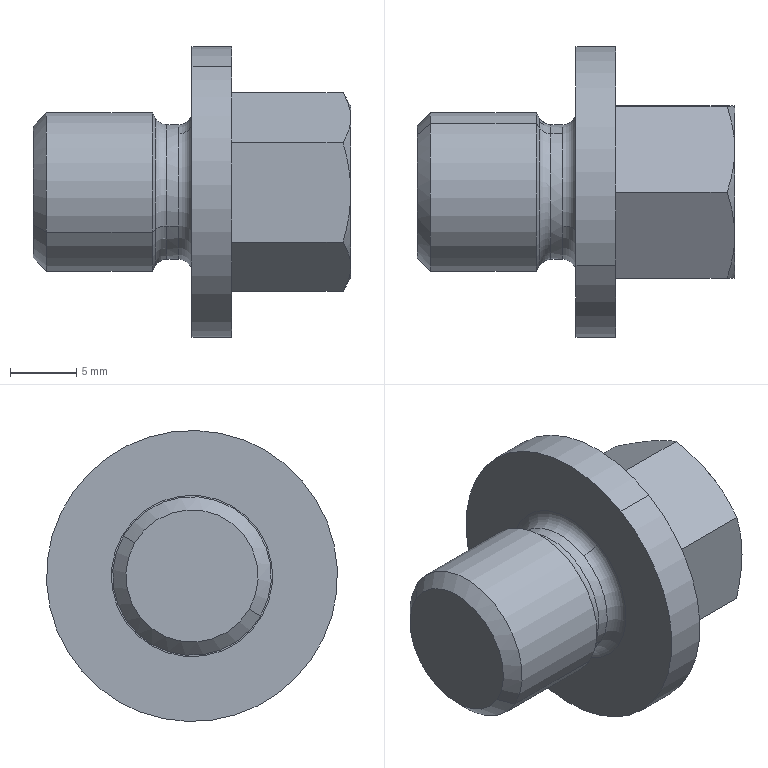Component | SolidWorks | JB_ZQ4450-1997[ExternalHexPlugM12_1.25]-1 | 1 solid | 30 faces | box 24 x 22 x 22 mm | volume 3717 mm3 | cone 10 | plane 10 | cylinder 6 | torus 4 | commonest cylinder face diameters 10.2 x2 12 x2 22 x2
STEP:
#1=COLOUR_RGB('',0.7922,0.8196,0.9333);
#2=FILL_AREA_STYLE_COLOUR('',#1);
#3=FILL_AREA_STYLE('',(#2));
#4=SURFACE_STYLE_FILL_AREA(#3);
#5=SURFACE_SIDE_STYLE('',(#4));
#6=SURFACE_STYLE_USAGE(.BOTH.,#5);
#7=PRESENTATION_STYLE_ASSIGNMENT((#6));
#8=CARTESIAN_POINT('',(7.835,-7.143,-0.1734));
#9=VERTEX_POINT('',#8);
#10=CARTESIAN_POINT('',(7.835,-7.417,-0.1013));
#11=VERTEX_POINT('',#10);
#12=CARTESIAN_POINT('',(7.835,-7.244,0.));
#13=DIRECTION('',(-1.,0.,0.));
#14=DIRECTION('',(0.,-0.5044,0.8635));
#15=AXIS2_PLACEMENT_3D('',#12,#13,#14);
#16=CIRCLE('',#15,0.2008);
#17=EDGE_CURVE('',#9,#11,#16,.T.);
#18=ORIENTED_EDGE('',*,*,#17,.F.);
#19=CARTESIAN_POINT('',(7.874,-7.123,-0.2074));
#20=VERTEX_POINT('',#19);
#21=CARTESIAN_POINT('',(7.835,-7.123,-0.2074));
#22=DIRECTION('',(0.,0.8635,0.5044));
#23=DIRECTION('',(0.,-0.5044,0.8635));
#24=AXIS2_PLACEMENT_3D('',#21,#22,#23);
#25=CIRCLE('',#24,0.03937);
#26=EDGE_CURVE('',#9,#20,#25,.T.);
#27=ORIENTED_EDGE('',*,*,#26,.T.);
#28=CARTESIAN_POINT('',(7.874,-7.365,0.2074));
#29=VERTEX_POINT('',#28);
#30=CARTESIAN_POINT('',(7.874,-7.244,0.));
#31=DIRECTION('',(1.,-0.,-0.));
#32=DIRECTION('',(0.,-0.5044,0.8635));
#33=AXIS2_PLACEMENT_3D('',#30,#31,#32);
#34=CIRCLE('',#33,0.2402);
#35=EDGE_CURVE('',#29,#20,#34,.T.);
#36=ORIENTED_EDGE('',*,*,#35,.F.);
#37=CARTESIAN_POINT('',(7.835,-7.345,0.1734));
#38=VERTEX_POINT('',#37);
#39=CARTESIAN_POINT('',(7.835,-7.365,0.2074));
#40=DIRECTION('',(-0.,-0.8635,-0.5044));
#41=DIRECTION('',(0.,0.5044,-0.8635));
#42=AXIS2_PLACEMENT_3D('',#39,#40,#41);
#43=CIRCLE('',#42,0.03937);
#44=EDGE_CURVE('',#38,#29,#43,.T.);
#45=ORIENTED_EDGE('',*,*,#44,.F.);
#46=CARTESIAN_POINT('',(7.835,-7.244,0.));
#47=DIRECTION('',(-1.,0.,0.));
#48=DIRECTION('',(0.,-0.5044,0.8635));
#49=AXIS2_PLACEMENT_3D('',#46,#47,#48);
#50=CIRCLE('',#49,0.2008);
#51=EDGE_CURVE('',#11,#38,#50,.T.);
#52=ORIENTED_EDGE('',*,*,#51,.F.);
#53=EDGE_LOOP('',(#18,#27,#36,#45,#52));
#54=FACE_OUTER_BOUND('',#53,.T.);
#55=CARTESIAN_POINT('',(7.835,-7.244,0.));
#56=DIRECTION('',(-1.,0.,0.));
#57=DIRECTION('',(-0.,-0.5044,0.8635));
#58=AXIS2_PLACEMENT_3D('',#55,#56,#57);
#59=TOROIDAL_SURFACE('',#58,0.2402,0.03937);
#60=ADVANCED_FACE('',(#54),#59,.F.);
#61=CARTESIAN_POINT('',(7.799,-7.417,-0.1013));
#62=VERTEX_POINT('',#61);
#63=CARTESIAN_POINT('',(7.799,-7.071,0.1013));
#64=VERTEX_POINT('',#63);
#65=CARTESIAN_POINT('',(7.799,-7.244,0.));
#66=DIRECTION('',(1.,-0.,0.));
#67=DIRECTION('',(0.,0.8635,0.5044));
#68=AXIS2_PLACEMENT_3D('',#65,#66,#67);
#69=CIRCLE('',#68,0.2008);
#70=EDGE_CURVE('',#62,#64,#69,.T.);
#71=ORIENTED_EDGE('',*,*,#70,.F.);
#72=CARTESIAN_POINT('',(7.765,-7.434,-0.1112));
#73=VERTEX_POINT('',#72);
#74=CARTESIAN_POINT('',(7.799,-7.451,-0.1211));
#75=DIRECTION('',(-0.,-0.5044,0.8635));
#76=DIRECTION('',(0.,-0.8635,-0.5044));
#77=AXIS2_PLACEMENT_3D('',#74,#75,#76);
#78=CIRCLE('',#77,0.03937);
#79=EDGE_CURVE('',#62,#73,#78,.T.);
#80=ORIENTED_EDGE('',*,*,#79,.T.);
#81=CARTESIAN_POINT('',(7.765,-7.054,0.1112));
#82=VERTEX_POINT('',#81);
#83=CARTESIAN_POINT('',(7.765,-7.244,0.));
#84=DIRECTION('',(-1.,0.,-0.));
#85=DIRECTION('',(0.,-0.8635,-0.5044));
#86=AXIS2_PLACEMENT_3D('',#83,#84,#85);
#87=CIRCLE('',#86,0.2205);
#88=EDGE_CURVE('',#82,#73,#87,.T.);
#89=ORIENTED_EDGE('',*,*,#88,.F.);
#90=CARTESIAN_POINT('',(7.799,-7.037,0.1211));
#91=DIRECTION('',(0.,0.5044,-0.8635));
#92=DIRECTION('',(0.,0.8635,0.5044));
#93=AXIS2_PLACEMENT_3D('',#90,#91,#92);
#94=CIRCLE('',#93,0.03937);
#95=EDGE_CURVE('',#64,#82,#94,.T.);
#96=ORIENTED_EDGE('',*,*,#95,.F.);
#97=EDGE_LOOP('',(#71,#80,#89,#96));
#98=FACE_OUTER_BOUND('',#97,.T.);
#99=CARTESIAN_POINT('',(7.799,-7.244,0.));
#100=DIRECTION('',(1.,-0.,0.));
#101=DIRECTION('',(0.,0.8635,0.5044));
#102=AXIS2_PLACEMENT_3D('',#99,#100,#101);
#103=TOROIDAL_SURFACE('',#102,0.2402,0.03937);
#104=ADVANCED_FACE('',(#98),#103,.F.);
#105=CARTESIAN_POINT('',(7.799,-7.244,0.));
#106=DIRECTION('',(1.,-0.,0.));
#107=DIRECTION('',(0.,0.8635,0.5044));
#108=AXIS2_PLACEMENT_3D('',#105,#106,#107);
#109=CIRCLE('',#108,0.2008);
#110=EDGE_CURVE('',#64,#62,#109,.T.);
#111=ORIENTED_EDGE('',*,*,#110,.T.);
#112=CARTESIAN_POINT('',(8.346,-7.417,-0.1013));
#113=DIRECTION('',(1.,-0.,0.));
#114=VECTOR('',#113,39.37);
#115=LINE('',#112,#114);
#116=EDGE_CURVE('',#62,#11,#115,.T.);
#117=ORIENTED_EDGE('',*,*,#116,.T.);
#118=ORIENTED_EDGE('',*,*,#51,.T.);
#119=CARTESIAN_POINT('',(7.835,-7.071,0.1013));
#120=VERTEX_POINT('',#119);
#121=CARTESIAN_POINT('',(7.835,-7.244,0.));
#122=DIRECTION('',(-1.,0.,0.));
#123=DIRECTION('',(0.,-0.5044,0.8635));
#124=AXIS2_PLACEMENT_3D('',#121,#122,#123);
#125=CIRCLE('',#124,0.2008);
#126=EDGE_CURVE('',#38,#120,#125,.T.);
#127=ORIENTED_EDGE('',*,*,#126,.T.);
#128=CARTESIAN_POINT('',(8.346,-7.071,0.1013));
#129=DIRECTION('',(1.,-0.,0.));
#130=VECTOR('',#129,39.37);
#131=LINE('',#128,#130);
#132=EDGE_CURVE('',#64,#120,#131,.T.);
#133=ORIENTED_EDGE('',*,*,#132,.F.);
#134=EDGE_LOOP('',(#111,#117,#118,#127,#133));
#135=FACE_OUTER_BOUND('',#134,.T.);
#136=CARTESIAN_POINT('',(8.346,-7.244,0.));
#137=DIRECTION('',(1.,-0.,0.));
#138=DIRECTION('',(0.,0.8635,0.5044));
#139=AXIS2_PLACEMENT_3D('',#136,#137,#138);
#140=CYLINDRICAL_SURFACE('',#139,0.2008);
#141=ADVANCED_FACE('',(#135),#140,.T.);
#142=CARTESIAN_POINT('',(7.765,-7.244,0.));
#143=DIRECTION('',(-1.,0.,-0.));
#144=DIRECTION('',(0.,-0.8635,-0.5044));
#145=AXIS2_PLACEMENT_3D('',#142,#143,#144);
#146=CIRCLE('',#145,0.2205);
#147=EDGE_CURVE('',#73,#82,#146,.T.);
#148=ORIENTED_EDGE('',*,*,#147,.T.);
#149=CARTESIAN_POINT('',(7.756,-7.04,0.1192));
#150=VERTEX_POINT('',#149);
#151=CARTESIAN_POINT('',(7.776,-7.071,0.1013));
#152=DIRECTION('',(-0.5,0.7478,0.4368));
#153=VECTOR('',#152,39.37);
#154=LINE('',#151,#153);
#155=EDGE_CURVE('',#82,#150,#154,.T.);
#156=ORIENTED_EDGE('',*,*,#155,.T.);
#157=CARTESIAN_POINT('',(7.756,-7.448,-0.1192));
#158=VERTEX_POINT('',#157);
#159=CARTESIAN_POINT('',(7.756,-7.244,0.));
#160=DIRECTION('',(1.,-0.,0.));
#161=DIRECTION('',(0.,0.8635,0.5044));
#162=AXIS2_PLACEMENT_3D('',#159,#160,#161);
#163=CIRCLE('',#162,0.2362);
#164=EDGE_CURVE('',#150,#158,#163,.T.);
#165=ORIENTED_EDGE('',*,*,#164,.T.);
#166=CARTESIAN_POINT('',(7.776,-7.417,-0.1013));
#167=DIRECTION('',(-0.5,-0.7478,-0.4368));
#168=VECTOR('',#167,39.37);
#169=LINE('',#166,#168);
#170=EDGE_CURVE('',#73,#158,#169,.T.);
#171=ORIENTED_EDGE('',*,*,#170,.F.);
#172=EDGE_LOOP('',(#148,#156,#165,#171));
#173=FACE_OUTER_BOUND('',#172,.T.);
#174=CARTESIAN_POINT('',(7.776,-7.244,0.));
#175=DIRECTION('',(-1.,0.,-0.));
#176=DIRECTION('',(0.,-0.8635,-0.5044));
#177=AXIS2_PLACEMENT_3D('',#174,#175,#176);
#178=CONICAL_SURFACE('',#177,0.2008,1.047);
#179=ADVANCED_FACE('',(#173),#178,.T.);
#180=CARTESIAN_POINT('',(7.441,-7.04,0.1192));
#181=VERTEX_POINT('',#180);
#182=CARTESIAN_POINT('',(7.441,-7.448,-0.1192));
#183=VERTEX_POINT('',#182);
#184=CARTESIAN_POINT('',(7.441,-7.244,0.));
#185=DIRECTION('',(1.,-0.,0.));
#186=DIRECTION('',(0.,0.8635,0.5044));
#187=AXIS2_PLACEMENT_3D('',#184,#185,#186);
#188=CIRCLE('',#187,0.2362);
#189=EDGE_CURVE('',#181,#183,#188,.T.);
#190=ORIENTED_EDGE('',*,*,#189,.T.);
#191=CARTESIAN_POINT('',(8.346,-7.448,-0.1192));
#192=DIRECTION('',(1.,-0.,0.));
#193=VECTOR('',#192,39.37);
#194=LINE('',#191,#193);
#195=EDGE_CURVE('',#183,#158,#194,.T.);
#196=ORIENTED_EDGE('',*,*,#195,.T.);
#197=ORIENTED_EDGE('',*,*,#164,.F.);
#198=CARTESIAN_POINT('',(8.346,-7.04,0.1192));
#199=DIRECTION('',(1.,-0.,0.));
#200=VECTOR('',#199,39.37);
#201=LINE('',#198,#200);
#202=EDGE_CURVE('',#181,#150,#201,.T.);
#203=ORIENTED_EDGE('',*,*,#202,.F.);
#204=EDGE_LOOP('',(#190,#196,#197,#203));
#205=FACE_OUTER_BOUND('',#204,.T.);
#206=CARTESIAN_POINT('',(8.346,-7.244,0.));
#207=DIRECTION('',(1.,-0.,0.));
#208=DIRECTION('',(0.,0.8635,0.5044));
#209=AXIS2_PLACEMENT_3D('',#206,#207,#208);
#210=CYLINDRICAL_SURFACE('',#209,0.2362);
#211=ADVANCED_FACE('',(#205),#210,.T.);
#212=CARTESIAN_POINT('',(7.402,-7.074,0.09929));
#213=VERTEX_POINT('',#212);
#214=CARTESIAN_POINT('',(7.402,-7.414,-0.09929));
#215=VERTEX_POINT('',#214);
#216=CARTESIAN_POINT('',(7.402,-7.244,0.));
#217=DIRECTION('',(1.,-0.,0.));
#218=DIRECTION('',(0.,0.8635,0.5044));
#219=AXIS2_PLACEMENT_3D('',#216,#217,#218);
#220=CIRCLE('',#219,0.1969);
#221=EDGE_CURVE('',#213,#215,#220,.T.);
#222=ORIENTED_EDGE('',*,*,#221,.T.);
#223=CARTESIAN_POINT('',(7.441,-7.448,-0.1192));
#224=DIRECTION('',(0.7071,-0.6106,-0.3567));
#225=VECTOR('',#224,39.37);
#226=LINE('',#223,#225);
#227=EDGE_CURVE('',#215,#183,#226,.T.);
#228=ORIENTED_EDGE('',*,*,#227,.T.);
#229=ORIENTED_EDGE('',*,*,#189,.F.);
#230=CARTESIAN_POINT('',(7.441,-7.04,0.1192));
#231=DIRECTION('',(0.7071,0.6106,0.3567));
#232=VECTOR('',#231,39.37);
#233=LINE('',#230,#232);
#234=EDGE_CURVE('',#213,#181,#233,.T.);
#235=ORIENTED_EDGE('',*,*,#234,.F.);
#236=EDGE_LOOP('',(#222,#228,#229,#235));
#237=FACE_OUTER_BOUND('',#236,.T.);
#238=CARTESIAN_POINT('',(7.441,-7.244,0.));
#239=DIRECTION('',(1.,-0.,0.));
#240=DIRECTION('',(0.,0.8635,0.5044));
#241=AXIS2_PLACEMENT_3D('',#238,#239,#240);
#242=CONICAL_SURFACE('',#241,0.2362,0.7854);
#243=ADVANCED_FACE('',(#237),#242,.T.);
#244=CARTESIAN_POINT('',(7.992,-7.463,0.3739));
#245=VERTEX_POINT('',#244);
#246=CARTESIAN_POINT('',(7.992,-7.026,-0.3739));
#247=VERTEX_POINT('',#246);
#248=CARTESIAN_POINT('',(7.992,-7.244,0.));
#249=DIRECTION('',(-1.,0.,0.));
#250=DIRECTION('',(0.,-0.5044,0.8635));
#251=AXIS2_PLACEMENT_3D('',#248,#249,#250);
#252=CIRCLE('',#251,0.4331);
#253=EDGE_CURVE('',#245,#247,#252,.T.);
#254=ORIENTED_EDGE('',*,*,#253,.T.);
#255=CARTESIAN_POINT('',(7.874,-7.026,-0.3739));
#256=VERTEX_POINT('',#255);
#257=CARTESIAN_POINT('',(7.992,-7.026,-0.3739));
#258=DIRECTION('',(-1.,0.,0.));
#259=VECTOR('',#258,39.37);
#260=LINE('',#257,#259);
#261=EDGE_CURVE('',#247,#256,#260,.T.);
#262=ORIENTED_EDGE('',*,*,#261,.T.);
#263=CARTESIAN_POINT('',(7.874,-7.463,0.3739));
#264=VERTEX_POINT('',#263);
#265=CARTESIAN_POINT('',(7.874,-7.244,0.));
#266=DIRECTION('',(-1.,0.,0.));
#267=DIRECTION('',(0.,-0.5044,0.8635));
#268=AXIS2_PLACEMENT_3D('',#265,#266,#267);
#269=CIRCLE('',#268,0.4331);
#270=EDGE_CURVE('',#264,#256,#269,.T.);
#271=ORIENTED_EDGE('',*,*,#270,.F.);
#272=CARTESIAN_POINT('',(7.992,-7.463,0.3739));
#273=DIRECTION('',(-1.,0.,0.));
#274=VECTOR('',#273,39.37);
#275=LINE('',#272,#274);
#276=EDGE_CURVE('',#245,#264,#275,.T.);
#277=ORIENTED_EDGE('',*,*,#276,.F.);
#278=EDGE_LOOP('',(#254,#262,#271,#277));
#279=FACE_OUTER_BOUND('',#278,.T.);
#280=CARTESIAN_POINT('',(7.992,-7.244,0.));
#281=DIRECTION('',(-1.,0.,0.));
#282=DIRECTION('',(0.,-0.5044,0.8635));
#283=AXIS2_PLACEMENT_3D('',#280,#281,#282);
#284=CYLINDRICAL_SURFACE('',#283,0.4331);
#285=ADVANCED_FACE('',(#279),#284,.T.);
#286=CARTESIAN_POINT('',(8.324,-6.989,0.1491));
#287=VERTEX_POINT('',#286);
#288=CARTESIAN_POINT('',(8.346,-7.117,0.2223));
#289=VERTEX_POINT('',#288);
#290=CARTESIAN_POINT('',(8.324,-6.989,0.1491));
#291=CARTESIAN_POINT('',(8.331,-7.01,0.161));
#292=CARTESIAN_POINT('',(8.336,-7.031,0.1731));
#293=CARTESIAN_POINT('',(8.344,-7.074,0.1975));
#294=CARTESIAN_POINT('',(8.346,-7.095,0.2098));
#295=CARTESIAN_POINT('',(8.346,-7.117,0.2223));
#296=B_SPLINE_CURVE_WITH_KNOTS('',3,(#290,#291,#292,#293,#294,#295),.UNSPECIFIED.,.F.,.F.,(4,2,4),(0.00000024,0.001899,0.003797),.UNSPECIFIED.);
#297=EDGE_CURVE('',#287,#289,#296,.T.);
#298=ORIENTED_EDGE('',*,*,#297,.F.);
#299=CARTESIAN_POINT('',(7.992,-6.989,0.1491));
#300=VERTEX_POINT('',#299);
#301=CARTESIAN_POINT('',(7.874,-6.989,0.1491));
#302=DIRECTION('',(1.,-0.,-0.));
#303=VECTOR('',#302,39.37);
#304=LINE('',#301,#303);
#305=EDGE_CURVE('',#300,#287,#304,.T.);
#306=ORIENTED_EDGE('',*,*,#305,.F.);
#307=CARTESIAN_POINT('',(7.992,-7.246,0.2955));
#308=VERTEX_POINT('',#307);
#309=CARTESIAN_POINT('',(7.992,-7.246,0.2955));
#310=DIRECTION('',(0.,0.8686,-0.4956));
#311=VECTOR('',#310,39.37);
#312=LINE('',#309,#311);
#313=EDGE_CURVE('',#308,#300,#312,.T.);
#314=ORIENTED_EDGE('',*,*,#313,.F.);
#315=CARTESIAN_POINT('',(8.324,-7.246,0.2955));
#316=VERTEX_POINT('',#315);
#317=CARTESIAN_POINT('',(7.874,-7.246,0.2955));
#318=DIRECTION('',(1.,-0.,-0.));
#319=VECTOR('',#318,39.37);
#320=LINE('',#317,#319);
#321=EDGE_CURVE('',#308,#316,#320,.T.);
#322=ORIENTED_EDGE('',*,*,#321,.T.);
#323=CARTESIAN_POINT('',(8.346,-7.117,0.2223));
#324=CARTESIAN_POINT('',(8.346,-7.128,0.2285));
#325=CARTESIAN_POINT('',(8.346,-7.139,0.2347));
#326=CARTESIAN_POINT('',(8.344,-7.161,0.2471));
#327=CARTESIAN_POINT('',(8.342,-7.171,0.2532));
#328=CARTESIAN_POINT('',(8.336,-7.204,0.2715));
#329=CARTESIAN_POINT('',(8.331,-7.225,0.2835));
#330=CARTESIAN_POINT('',(8.324,-7.246,0.2955));
#331=B_SPLINE_CURVE_WITH_KNOTS('',3,(#323,#324,#325,#326,#327,#328,#329,#330),.UNSPECIFIED.,.F.,.F.,(4,2,2,4),(0.003797,0.004743,0.005689,0.00758),.UNSPECIFIED.);
#332=EDGE_CURVE('',#289,#316,#331,.T.);
#333=ORIENTED_EDGE('',*,*,#332,.F.);
#334=EDGE_LOOP('',(#298,#306,#314,#322,#333));
#335=FACE_OUTER_BOUND('',#334,.T.);
#336=CARTESIAN_POINT('',(7.874,-7.246,0.2955));
#337=DIRECTION('',(-0.,-0.4956,-0.8686));
#338=DIRECTION('',(-0.,-0.8686,0.4956));
#339=AXIS2_PLACEMENT_3D('',#336,#337,#338);
#340=PLANE('',#339);
#341=ADVANCED_FACE('',(#335),#340,.F.);
#342=CARTESIAN_POINT('',(8.324,-6.987,-0.1464));
#343=VERTEX_POINT('',#342);
#344=CARTESIAN_POINT('',(8.346,-6.988,0.001305));
#345=VERTEX_POINT('',#344);
#346=CARTESIAN_POINT('',(8.324,-6.987,-0.1464));
#347=CARTESIAN_POINT('',(8.331,-6.988,-0.1223));
#348=CARTESIAN_POINT('',(8.336,-6.988,-0.09793));
#349=CARTESIAN_POINT('',(8.344,-6.988,-0.04872));
#350=CARTESIAN_POINT('',(8.346,-6.988,-0.02387));
#351=CARTESIAN_POINT('',(8.346,-6.988,0.001305));
#352=B_SPLINE_CURVE_WITH_KNOTS('',3,(#346,#347,#348,#349,#350,#351),.UNSPECIFIED.,.F.,.F.,(4,2,4),(0.00000024,0.001899,0.003797),.UNSPECIFIED.);
#353=EDGE_CURVE('',#343,#345,#352,.T.);
#354=ORIENTED_EDGE('',*,*,#353,.F.);
#355=CARTESIAN_POINT('',(7.992,-6.987,-0.1464));
#356=VERTEX_POINT('',#355);
#357=CARTESIAN_POINT('',(7.874,-6.987,-0.1464));
#358=DIRECTION('',(1.,-0.,-0.));
#359=VECTOR('',#358,39.37);
#360=LINE('',#357,#359);
#361=EDGE_CURVE('',#356,#343,#360,.T.);
#362=ORIENTED_EDGE('',*,*,#361,.F.);
#363=CARTESIAN_POINT('',(7.992,-6.989,0.1491));
#364=DIRECTION('',(-0.,0.005099,-1.));
#365=VECTOR('',#364,39.37);
#366=LINE('',#363,#365);
#367=EDGE_CURVE('',#300,#356,#366,.T.);
#368=ORIENTED_EDGE('',*,*,#367,.F.);
#369=ORIENTED_EDGE('',*,*,#305,.T.);
#370=CARTESIAN_POINT('',(8.346,-6.988,0.001305));
#371=CARTESIAN_POINT('',(8.346,-6.988,0.01384));
#372=CARTESIAN_POINT('',(8.346,-6.988,0.02644));
#373=CARTESIAN_POINT('',(8.344,-6.988,0.05135));
#374=CARTESIAN_POINT('',(8.342,-6.989,0.06373));
#375=CARTESIAN_POINT('',(8.336,-6.989,0.1006));
#376=CARTESIAN_POINT('',(8.331,-6.989,0.1249));
#377=CARTESIAN_POINT('',(8.324,-6.989,0.1491));
#378=B_SPLINE_CURVE_WITH_KNOTS('',3,(#370,#371,#372,#373,#374,#375,#376,#377),.UNSPECIFIED.,.F.,.F.,(4,2,2,4),(0.003797,0.004743,0.005689,0.00758),.UNSPECIFIED.);
#379=EDGE_CURVE('',#345,#287,#378,.T.);
#380=ORIENTED_EDGE('',*,*,#379,.F.);
#381=EDGE_LOOP('',(#354,#362,#368,#369,#380));
#382=FACE_OUTER_BOUND('',#381,.T.);
#383=CARTESIAN_POINT('',(7.874,-6.989,0.1491));
#384=DIRECTION('',(-0.,-1.,-0.005099));
#385=DIRECTION('',(0.,-0.005099,1.));
#386=AXIS2_PLACEMENT_3D('',#383,#384,#385);
#387=PLANE('',#386);
#388=ADVANCED_FACE('',(#382),#387,.F.);
#389=CARTESIAN_POINT('',(8.324,-7.243,-0.2955));
#390=VERTEX_POINT('',#389);
#391=CARTESIAN_POINT('',(8.346,-7.115,-0.221));
#392=VERTEX_POINT('',#391);
#393=CARTESIAN_POINT('',(8.324,-7.243,-0.2955));
#394=CARTESIAN_POINT('',(8.331,-7.222,-0.2833));
#395=CARTESIAN_POINT('',(8.336,-7.201,-0.2709));
#396=CARTESIAN_POINT('',(8.344,-7.158,-0.2461));
#397=CARTESIAN_POINT('',(8.346,-7.137,-0.2336));
#398=CARTESIAN_POINT('',(8.346,-7.115,-0.221));
#399=B_SPLINE_CURVE_WITH_KNOTS('',3,(#393,#394,#395,#396,#397,#398),.UNSPECIFIED.,.F.,.F.,(4,2,4),(0.007073,0.008973,0.01087),.UNSPECIFIED.);
#400=EDGE_CURVE('',#390,#392,#399,.T.);
#401=ORIENTED_EDGE('',*,*,#400,.F.);
#402=CARTESIAN_POINT('',(7.992,-7.243,-0.2955));
#403=VERTEX_POINT('',#402);
#404=CARTESIAN_POINT('',(7.874,-7.243,-0.2955));
#405=DIRECTION('',(1.,-0.,-0.));
#406=VECTOR('',#405,39.37);
#407=LINE('',#404,#406);
#408=EDGE_CURVE('',#403,#390,#407,.T.);
#409=ORIENTED_EDGE('',*,*,#408,.F.);
#410=CARTESIAN_POINT('',(7.992,-6.987,-0.1464));
#411=DIRECTION('',(-0.,-0.8635,-0.5044));
#412=VECTOR('',#411,39.37);
#413=LINE('',#410,#412);
#414=EDGE_CURVE('',#356,#403,#413,.T.);
#415=ORIENTED_EDGE('',*,*,#414,.F.);
#416=ORIENTED_EDGE('',*,*,#361,.T.);
#417=CARTESIAN_POINT('',(8.346,-7.115,-0.221));
#418=CARTESIAN_POINT('',(8.346,-7.104,-0.2147));
#419=CARTESIAN_POINT('',(8.346,-7.093,-0.2083));
#420=CARTESIAN_POINT('',(8.344,-7.072,-0.1956));
#421=CARTESIAN_POINT('',(8.342,-7.061,-0.1893));
#422=CARTESIAN_POINT('',(8.336,-7.029,-0.1707));
#423=CARTESIAN_POINT('',(8.331,-7.008,-0.1585));
#424=CARTESIAN_POINT('',(8.324,-6.987,-0.1464));
#425=B_SPLINE_CURVE_WITH_KNOTS('',3,(#417,#418,#419,#420,#421,#422,#423,#424),.UNSPECIFIED.,.F.,.F.,(4,2,2,4),(0.01087,0.01182,0.01277,0.01468),.UNSPECIFIED.);
#426=EDGE_CURVE('',#392,#343,#425,.T.);
#427=ORIENTED_EDGE('',*,*,#426,.F.);
#428=EDGE_LOOP('',(#401,#409,#415,#416,#427));
#429=FACE_OUTER_BOUND('',#428,.T.);
#430=CARTESIAN_POINT('',(7.874,-6.987,-0.1464));
#431=DIRECTION('',(-0.,-0.5044,0.8635));
#432=DIRECTION('',(0.,0.8635,0.5044));
#433=AXIS2_PLACEMENT_3D('',#430,#431,#432);
#434=PLANE('',#433);
#435=ADVANCED_FACE('',(#429),#434,.F.);
#436=CARTESIAN_POINT('',(8.324,-7.499,-0.1491));
#437=VERTEX_POINT('',#436);
#438=CARTESIAN_POINT('',(8.346,-7.371,-0.2223));
#439=VERTEX_POINT('',#438);
#440=CARTESIAN_POINT('',(8.324,-7.499,-0.1491));
#441=CARTESIAN_POINT('',(8.331,-7.478,-0.161));
#442=CARTESIAN_POINT('',(8.336,-7.457,-0.1731));
#443=CARTESIAN_POINT('',(8.344,-7.414,-0.1975));
#444=CARTESIAN_POINT('',(8.346,-7.393,-0.2098));
#445=CARTESIAN_POINT('',(8.346,-7.371,-0.2223));
#446=B_SPLINE_CURVE_WITH_KNOTS('',3,(#440,#441,#442,#443,#444,#445),.UNSPECIFIED.,.F.,.F.,(4,2,4),(0.00000024,0.001899,0.003797),.UNSPECIFIED.);
#447=EDGE_CURVE('',#437,#439,#446,.T.);
#448=ORIENTED_EDGE('',*,*,#447,.F.);
#449=CARTESIAN_POINT('',(7.992,-7.499,-0.1491));
#450=VERTEX_POINT('',#449);
#451=CARTESIAN_POINT('',(7.874,-7.499,-0.1491));
#452=DIRECTION('',(1.,-0.,-0.));
#453=VECTOR('',#452,39.37);
#454=LINE('',#451,#453);
#455=EDGE_CURVE('',#450,#437,#454,.T.);
#456=ORIENTED_EDGE('',*,*,#455,.F.);
#457=CARTESIAN_POINT('',(7.992,-7.243,-0.2955));
#458=DIRECTION('',(-0.,-0.8686,0.4956));
#459=VECTOR('',#458,39.37);
#460=LINE('',#457,#459);
#461=EDGE_CURVE('',#403,#450,#460,.T.);
#462=ORIENTED_EDGE('',*,*,#461,.F.);
#463=ORIENTED_EDGE('',*,*,#408,.T.);
#464=CARTESIAN_POINT('',(8.346,-7.371,-0.2223));
#465=CARTESIAN_POINT('',(8.346,-7.36,-0.2285));
#466=CARTESIAN_POINT('',(8.346,-7.349,-0.2347));
#467=CARTESIAN_POINT('',(8.344,-7.327,-0.2471));
#468=CARTESIAN_POINT('',(8.342,-7.317,-0.2532));
#469=CARTESIAN_POINT('',(8.336,-7.285,-0.2715));
#470=CARTESIAN_POINT('',(8.331,-7.264,-0.2835));
#471=CARTESIAN_POINT('',(8.324,-7.243,-0.2955));
#472=B_SPLINE_CURVE_WITH_KNOTS('',3,(#464,#465,#466,#467,#468,#469,#470,#471),.UNSPECIFIED.,.F.,.F.,(4,2,2,4),(0.003797,0.004743,0.005689,0.00758),.UNSPECIFIED.);
#473=EDGE_CURVE('',#439,#390,#472,.T.);
#474=ORIENTED_EDGE('',*,*,#473,.F.);
#475=EDGE_LOOP('',(#448,#456,#462,#463,#474));
#476=FACE_OUTER_BOUND('',#475,.T.);
#477=CARTESIAN_POINT('',(7.874,-7.243,-0.2955));
#478=DIRECTION('',(0.,0.4956,0.8686));
#479=DIRECTION('',(0.,0.8686,-0.4956));
#480=AXIS2_PLACEMENT_3D('',#477,#478,#479);
#481=PLANE('',#480);
#482=ADVANCED_FACE('',(#476),#481,.F.);
#483=CARTESIAN_POINT('',(8.324,-7.501,0.1464));
#484=VERTEX_POINT('',#483);
#485=CARTESIAN_POINT('',(8.346,-7.5,-0.001305));
#486=VERTEX_POINT('',#485);
#487=CARTESIAN_POINT('',(8.324,-7.501,0.1464));
#488=CARTESIAN_POINT('',(8.331,-7.501,0.1223));
#489=CARTESIAN_POINT('',(8.336,-7.501,0.09793));
#490=CARTESIAN_POINT('',(8.344,-7.5,0.04872));
#491=CARTESIAN_POINT('',(8.346,-7.5,0.02387));
#492=CARTESIAN_POINT('',(8.346,-7.5,-0.001305));
#493=B_SPLINE_CURVE_WITH_KNOTS('',3,(#487,#488,#489,#490,#491,#492),.UNSPECIFIED.,.F.,.F.,(4,2,4),(0.00000024,0.001899,0.003797),.UNSPECIFIED.);
#494=EDGE_CURVE('',#484,#486,#493,.T.);
#495=ORIENTED_EDGE('',*,*,#494,.F.);
#496=CARTESIAN_POINT('',(7.992,-7.501,0.1464));
#497=VERTEX_POINT('',#496);
#498=CARTESIAN_POINT('',(7.874,-7.501,0.1464));
#499=DIRECTION('',(1.,-0.,-0.));
#500=VECTOR('',#499,39.37);
#501=LINE('',#498,#500);
#502=EDGE_CURVE('',#497,#484,#501,.T.);
#503=ORIENTED_EDGE('',*,*,#502,.F.);
#504=CARTESIAN_POINT('',(7.992,-7.499,-0.1491));
#505=DIRECTION('',(0.,-0.005099,1.));
#506=VECTOR('',#505,39.37);
#507=LINE('',#504,#506);
#508=EDGE_CURVE('',#450,#497,#507,.T.);
#509=ORIENTED_EDGE('',*,*,#508,.F.);
#510=ORIENTED_EDGE('',*,*,#455,.T.);
#511=CARTESIAN_POINT('',(8.346,-7.5,-0.001305));
#512=CARTESIAN_POINT('',(8.346,-7.5,-0.01384));
#513=CARTESIAN_POINT('',(8.346,-7.5,-0.02644));
#514=CARTESIAN_POINT('',(8.344,-7.5,-0.05135));
#515=CARTESIAN_POINT('',(8.342,-7.5,-0.06373));
#516=CARTESIAN_POINT('',(8.336,-7.499,-0.1006));
#517=CARTESIAN_POINT('',(8.331,-7.499,-0.1249));
#518=CARTESIAN_POINT('',(8.324,-7.499,-0.1491));
#519=B_SPLINE_CURVE_WITH_KNOTS('',3,(#511,#512,#513,#514,#515,#516,#517,#518),.UNSPECIFIED.,.F.,.F.,(4,2,2,4),(0.003797,0.004743,0.005689,0.00758),.UNSPECIFIED.);
#520=EDGE_CURVE('',#486,#437,#519,.T.);
#521=ORIENTED_EDGE('',*,*,#520,.F.);
#522=EDGE_LOOP('',(#495,#503,#509,#510,#521));
#523=FACE_OUTER_BOUND('',#522,.T.);
#524=CARTESIAN_POINT('',(7.874,-7.499,-0.1491));
#525=DIRECTION('',(0.,1.,0.005099));
#526=DIRECTION('',(-0.,0.005099,-1.));
#527=AXIS2_PLACEMENT_3D('',#524,#525,#526);
#528=PLANE('',#527);
#529=ADVANCED_FACE('',(#523),#528,.F.);
#530=CARTESIAN_POINT('',(8.346,-7.373,0.221));
#531=VERTEX_POINT('',#530);
#532=CARTESIAN_POINT('',(8.324,-7.246,0.2955));
#533=CARTESIAN_POINT('',(8.331,-7.266,0.2834));
#534=CARTESIAN_POINT('',(8.336,-7.287,0.2712));
#535=CARTESIAN_POINT('',(8.342,-7.319,0.2526));
#536=CARTESIAN_POINT('',(8.344,-7.33,0.2463));
#537=CARTESIAN_POINT('',(8.346,-7.351,0.2336));
#538=CARTESIAN_POINT('',(8.346,-7.362,0.2273));
#539=CARTESIAN_POINT('',(8.346,-7.373,0.221));
#540=B_SPLINE_CURVE_WITH_KNOTS('',3,(#532,#533,#534,#535,#536,#537,#538,#539),.UNSPECIFIED.,.F.,.F.,(4,2,2,4),(0.01868,0.02058,0.02153,0.02248),.UNSPECIFIED.);
#541=EDGE_CURVE('',#316,#531,#540,.T.);
#542=ORIENTED_EDGE('',*,*,#541,.F.);
#543=ORIENTED_EDGE('',*,*,#321,.F.);
#544=CARTESIAN_POINT('',(7.992,-7.501,0.1464));
#545=DIRECTION('',(0.,0.8635,0.5044));
#546=VECTOR('',#545,39.37);
#547=LINE('',#544,#546);
#548=EDGE_CURVE('',#497,#308,#547,.T.);
#549=ORIENTED_EDGE('',*,*,#548,.F.);
#550=ORIENTED_EDGE('',*,*,#502,.T.);
#551=CARTESIAN_POINT('',(8.346,-7.373,0.221));
#552=CARTESIAN_POINT('',(8.346,-7.395,0.2083));
#553=CARTESIAN_POINT('',(8.344,-7.416,0.1958));
#554=CARTESIAN_POINT('',(8.336,-7.459,0.171));
#555=CARTESIAN_POINT('',(8.331,-7.48,0.1586));
#556=CARTESIAN_POINT('',(8.324,-7.501,0.1464));
#557=B_SPLINE_CURVE_WITH_KNOTS('',3,(#551,#552,#553,#554,#555,#556),.UNSPECIFIED.,.F.,.F.,(4,2,4),(0.02248,0.02438,0.02628),.UNSPECIFIED.);
#558=EDGE_CURVE('',#531,#484,#557,.T.);
#559=ORIENTED_EDGE('',*,*,#558,.F.);
#560=EDGE_LOOP('',(#542,#543,#549,#550,#559));
#561=FACE_OUTER_BOUND('',#560,.T.);
#562=CARTESIAN_POINT('',(7.874,-7.501,0.1464));
#563=DIRECTION('',(0.,0.5044,-0.8635));
#564=DIRECTION('',(-0.,-0.8635,-0.5044));
#565=AXIS2_PLACEMENT_3D('',#562,#563,#564);
#566=PLANE('',#565);
#567=ADVANCED_FACE('',(#561),#566,.F.);
#568=ORIENTED_EDGE('',*,*,#253,.F.);
#569=CARTESIAN_POINT('',(7.992,-7.244,0.));
#570=DIRECTION('',(-1.,0.,0.));
#571=DIRECTION('',(0.,-0.5044,0.8635));
#572=AXIS2_PLACEMENT_3D('',#569,#570,#571);
#573=CIRCLE('',#572,0.4331);
#574=EDGE_CURVE('',#247,#245,#573,.T.);
#575=ORIENTED_EDGE('',*,*,#574,.F.);
#576=EDGE_LOOP('',(#568,#575));
#577=FACE_OUTER_BOUND('',#576,.T.);
#578=ORIENTED_EDGE('',*,*,#548,.T.);
#579=ORIENTED_EDGE('',*,*,#313,.T.);
#580=ORIENTED_EDGE('',*,*,#367,.T.);
#581=ORIENTED_EDGE('',*,*,#414,.T.);
#582=ORIENTED_EDGE('',*,*,#461,.T.);
#583=ORIENTED_EDGE('',*,*,#508,.T.);
#584=EDGE_LOOP('',(#578,#579,#580,#581,#582,#583));
#585=FACE_BOUND('',#584,.T.);
#586=CARTESIAN_POINT('',(7.992,-7.244,0.));
#587=DIRECTION('',(-1.,0.,0.));
#588=DIRECTION('',(-0.,-0.5044,0.8635));
#589=AXIS2_PLACEMENT_3D('',#586,#587,#588);
#590=PLANE('',#589);
#591=ADVANCED_FACE('',(#577,#585),#590,.F.);
#592=ORIENTED_EDGE('',*,*,#261,.F.);
#593=ORIENTED_EDGE('',*,*,#574,.T.);
#594=ORIENTED_EDGE('',*,*,#276,.T.);
#595=CARTESIAN_POINT('',(7.874,-7.244,0.));
#596=DIRECTION('',(-1.,0.,0.));
#597=DIRECTION('',(0.,-0.5044,0.8635));
#598=AXIS2_PLACEMENT_3D('',#595,#596,#597);
#599=CIRCLE('',#598,0.4331);
#600=EDGE_CURVE('',#256,#264,#599,.T.);
#601=ORIENTED_EDGE('',*,*,#600,.F.);
#602=EDGE_LOOP('',(#592,#593,#594,#601));
#603=FACE_OUTER_BOUND('',#602,.T.);
#604=CARTESIAN_POINT('',(7.992,-7.244,0.));
#605=DIRECTION('',(-1.,0.,0.));
#606=DIRECTION('',(0.,-0.5044,0.8635));
#607=AXIS2_PLACEMENT_3D('',#604,#605,#606);
#608=CYLINDRICAL_SURFACE('',#607,0.4331);
#609=ADVANCED_FACE('',(#603),#608,.T.);
#610=ORIENTED_EDGE('',*,*,#35,.T.);
#611=CARTESIAN_POINT('',(7.874,-7.244,0.));
#612=DIRECTION('',(1.,-0.,-0.));
#613=DIRECTION('',(0.,-0.5044,0.8635));
#614=AXIS2_PLACEMENT_3D('',#611,#612,#613);
#615=CIRCLE('',#614,0.2402);
#616=EDGE_CURVE('',#20,#29,#615,.T.);
#617=ORIENTED_EDGE('',*,*,#616,.T.);
#618=EDGE_LOOP('',(#610,#617));
#619=FACE_BOUND('',#618,.T.);
#620=ORIENTED_EDGE('',*,*,#270,.T.);
#621=ORIENTED_EDGE('',*,*,#600,.T.);
#622=EDGE_LOOP('',(#620,#621));
#623=FACE_OUTER_BOUND('',#622,.T.);
#624=CARTESIAN_POINT('',(7.874,-6.732,0.00261));
#625=DIRECTION('',(-1.,0.,0.));
#626=DIRECTION('',(-0.,-0.5044,0.8635));
#627=AXIS2_PLACEMENT_3D('',#624,#625,#626);
#628=PLANE('',#627);
#629=ADVANCED_FACE('',(#619,#623),#628,.T.);
#630=ORIENTED_EDGE('',*,*,#494,.T.);
#631=CARTESIAN_POINT('',(8.346,-7.244,0.));
#632=DIRECTION('',(-1.,0.,0.));
#633=DIRECTION('',(0.,-0.5044,0.8635));
#634=AXIS2_PLACEMENT_3D('',#631,#632,#633);
#635=CIRCLE('',#634,0.2559);
#636=EDGE_CURVE('',#486,#531,#635,.T.);
#637=ORIENTED_EDGE('',*,*,#636,.T.);
#638=ORIENTED_EDGE('',*,*,#558,.T.);
#639=EDGE_LOOP('',(#630,#637,#638));
#640=FACE_OUTER_BOUND('',#639,.T.);
#641=CARTESIAN_POINT('',(8.346,-7.244,0.));
#642=DIRECTION('',(-1.,0.,0.));
#643=DIRECTION('',(0.,0.5044,-0.8635));
#644=AXIS2_PLACEMENT_3D('',#641,#642,#643);
#645=CONICAL_SURFACE('',#644,0.2559,1.047);
#646=ADVANCED_FACE('',(#640),#645,.T.);
#647=ORIENTED_EDGE('',*,*,#447,.T.);
#648=CARTESIAN_POINT('',(8.346,-7.244,0.));
#649=DIRECTION('',(-1.,0.,0.));
#650=DIRECTION('',(0.,-0.5044,0.8635));
#651=AXIS2_PLACEMENT_3D('',#648,#649,#650);
#652=CIRCLE('',#651,0.2559);
#653=EDGE_CURVE('',#439,#486,#652,.T.);
#654=ORIENTED_EDGE('',*,*,#653,.T.);
#655=ORIENTED_EDGE('',*,*,#520,.T.);
#656=EDGE_LOOP('',(#647,#654,#655));
#657=FACE_OUTER_BOUND('',#656,.T.);
#658=CARTESIAN_POINT('',(8.346,-7.244,0.));
#659=DIRECTION('',(-1.,0.,0.));
#660=DIRECTION('',(0.,0.5044,-0.8635));
#661=AXIS2_PLACEMENT_3D('',#658,#659,#660);
#662=CONICAL_SURFACE('',#661,0.2559,1.047);
#663=ADVANCED_FACE('',(#657),#662,.T.);
#664=ORIENTED_EDGE('',*,*,#400,.T.);
#665=CARTESIAN_POINT('',(8.346,-7.244,0.));
#666=DIRECTION('',(-1.,0.,0.));
#667=DIRECTION('',(0.,-0.5044,0.8635));
#668=AXIS2_PLACEMENT_3D('',#665,#666,#667);
#669=CIRCLE('',#668,0.2559);
#670=EDGE_CURVE('',#392,#439,#669,.T.);
#671=ORIENTED_EDGE('',*,*,#670,.T.);
#672=ORIENTED_EDGE('',*,*,#473,.T.);
#673=EDGE_LOOP('',(#664,#671,#672));
#674=FACE_OUTER_BOUND('',#673,.T.);
#675=CARTESIAN_POINT('',(8.346,-7.244,0.));
#676=DIRECTION('',(-1.,0.,0.));
#677=DIRECTION('',(0.,0.5044,-0.8635));
#678=AXIS2_PLACEMENT_3D('',#675,#676,#677);
#679=CONICAL_SURFACE('',#678,0.2559,1.047);
#680=ADVANCED_FACE('',(#674),#679,.T.);
#681=ORIENTED_EDGE('',*,*,#426,.T.);
#682=ORIENTED_EDGE('',*,*,#353,.T.);
#683=CARTESIAN_POINT('',(8.346,-7.244,0.));
#684=DIRECTION('',(1.,-0.,-0.));
#685=DIRECTION('',(0.,0.5044,-0.8635));
#686=AXIS2_PLACEMENT_3D('',#683,#684,#685);
#687=CIRCLE('',#686,0.2559);
#688=EDGE_CURVE('',#392,#345,#687,.T.);
#689=ORIENTED_EDGE('',*,*,#688,.F.);
#690=EDGE_LOOP('',(#681,#682,#689));
#691=FACE_OUTER_BOUND('',#690,.T.);
#692=CARTESIAN_POINT('',(8.346,-7.244,0.));
#693=DIRECTION('',(-1.,0.,0.));
#694=DIRECTION('',(0.,0.5044,-0.8635));
#695=AXIS2_PLACEMENT_3D('',#692,#693,#694);
#696=CONICAL_SURFACE('',#695,0.2559,1.047);
#697=ADVANCED_FACE('',(#691),#696,.T.);
#698=ORIENTED_EDGE('',*,*,#379,.T.);
#699=ORIENTED_EDGE('',*,*,#297,.T.);
#700=CARTESIAN_POINT('',(8.346,-7.244,0.));
#701=DIRECTION('',(-1.,0.,0.));
#702=DIRECTION('',(0.,-0.5044,0.8635));
#703=AXIS2_PLACEMENT_3D('',#700,#701,#702);
#704=CIRCLE('',#703,0.2559);
#705=EDGE_CURVE('',#289,#345,#704,.T.);
#706=ORIENTED_EDGE('',*,*,#705,.T.);
#707=EDGE_LOOP('',(#698,#699,#706));
#708=FACE_OUTER_BOUND('',#707,.T.);
#709=CARTESIAN_POINT('',(8.346,-7.244,0.));
#710=DIRECTION('',(-1.,0.,0.));
#711=DIRECTION('',(0.,0.5044,-0.8635));
#712=AXIS2_PLACEMENT_3D('',#709,#710,#711);
#713=CONICAL_SURFACE('',#712,0.2559,1.047);
#714=ADVANCED_FACE('',(#708),#713,.T.);
#715=ORIENTED_EDGE('',*,*,#332,.T.);
#716=ORIENTED_EDGE('',*,*,#541,.T.);
#717=CARTESIAN_POINT('',(8.346,-7.244,0.));
#718=DIRECTION('',(-1.,0.,0.));
#719=DIRECTION('',(0.,-0.5044,0.8635));
#720=AXIS2_PLACEMENT_3D('',#717,#718,#719);
#721=CIRCLE('',#720,0.2559);
#722=EDGE_CURVE('',#531,#289,#721,.T.);
#723=ORIENTED_EDGE('',*,*,#722,.T.);
#724=EDGE_LOOP('',(#715,#716,#723));
#725=FACE_OUTER_BOUND('',#724,.T.);
#726=CARTESIAN_POINT('',(8.346,-7.244,0.));
#727=DIRECTION('',(-1.,0.,0.));
#728=DIRECTION('',(0.,0.5044,-0.8635));
#729=AXIS2_PLACEMENT_3D('',#726,#727,#728);
#730=CONICAL_SURFACE('',#729,0.2559,1.047);
#731=ADVANCED_FACE('',(#725),#730,.T.);
#732=ORIENTED_EDGE('',*,*,#722,.F.);
#733=ORIENTED_EDGE('',*,*,#636,.F.);
#734=ORIENTED_EDGE('',*,*,#653,.F.);
#735=ORIENTED_EDGE('',*,*,#670,.F.);
#736=ORIENTED_EDGE('',*,*,#688,.T.);
#737=ORIENTED_EDGE('',*,*,#705,.F.);
#738=EDGE_LOOP('',(#732,#733,#734,#735,#736,#737));
#739=FACE_OUTER_BOUND('',#738,.T.);
#740=CARTESIAN_POINT('',(8.346,-6.732,0.00261));
#741=DIRECTION('',(-1.,0.,0.));
#742=DIRECTION('',(-0.,-0.5044,0.8635));
#743=AXIS2_PLACEMENT_3D('',#740,#741,#742);
#744=PLANE('',#743);
#745=ADVANCED_FACE('',(#739),#744,.F.);
#746=ORIENTED_EDGE('',*,*,#221,.F.);
#747=CARTESIAN_POINT('',(7.402,-7.244,0.));
#748=DIRECTION('',(1.,-0.,0.));
#749=DIRECTION('',(0.,0.8635,0.5044));
#750=AXIS2_PLACEMENT_3D('',#747,#748,#749);
#751=CIRCLE('',#750,0.1969);
#752=EDGE_CURVE('',#215,#213,#751,.T.);
#753=ORIENTED_EDGE('',*,*,#752,.F.);
#754=EDGE_LOOP('',(#746,#753));
#755=FACE_OUTER_BOUND('',#754,.T.);
#756=CARTESIAN_POINT('',(7.402,-7.244,0.));
#757=DIRECTION('',(-1.,0.,-0.));
#758=DIRECTION('',(-0.,-0.8635,-0.5044));
#759=AXIS2_PLACEMENT_3D('',#756,#757,#758);
#760=PLANE('',#759);
#761=ADVANCED_FACE('',(#755),#760,.T.);
#762=ORIENTED_EDGE('',*,*,#227,.F.);
#763=ORIENTED_EDGE('',*,*,#752,.T.);
#764=ORIENTED_EDGE('',*,*,#234,.T.);
#765=CARTESIAN_POINT('',(7.441,-7.244,0.));
#766=DIRECTION('',(1.,-0.,0.));
#767=DIRECTION('',(0.,0.8635,0.5044));
#768=AXIS2_PLACEMENT_3D('',#765,#766,#767);
#769=CIRCLE('',#768,0.2362);
#770=EDGE_CURVE('',#183,#181,#769,.T.);
#771=ORIENTED_EDGE('',*,*,#770,.F.);
#772=EDGE_LOOP('',(#762,#763,#764,#771));
#773=FACE_OUTER_BOUND('',#772,.T.);
#774=CARTESIAN_POINT('',(7.441,-7.244,0.));
#775=DIRECTION('',(1.,-0.,0.));
#776=DIRECTION('',(0.,0.8635,0.5044));
#777=AXIS2_PLACEMENT_3D('',#774,#775,#776);
#778=CONICAL_SURFACE('',#777,0.2362,0.7854);
#779=ADVANCED_FACE('',(#773),#778,.T.);
#780=ORIENTED_EDGE('',*,*,#195,.F.);
#781=ORIENTED_EDGE('',*,*,#770,.T.);
#782=ORIENTED_EDGE('',*,*,#202,.T.);
#783=CARTESIAN_POINT('',(7.756,-7.244,0.));
#784=DIRECTION('',(1.,-0.,0.));
#785=DIRECTION('',(0.,0.8635,0.5044));
#786=AXIS2_PLACEMENT_3D('',#783,#784,#785);
#787=CIRCLE('',#786,0.2362);
#788=EDGE_CURVE('',#158,#150,#787,.T.);
#789=ORIENTED_EDGE('',*,*,#788,.F.);
#790=EDGE_LOOP('',(#780,#781,#782,#789));
#791=FACE_OUTER_BOUND('',#790,.T.);
#792=CARTESIAN_POINT('',(8.346,-7.244,0.));
#793=DIRECTION('',(1.,-0.,0.));
#794=DIRECTION('',(0.,0.8635,0.5044));
#795=AXIS2_PLACEMENT_3D('',#792,#793,#794);
#796=CYLINDRICAL_SURFACE('',#795,0.2362);
#797=ADVANCED_FACE('',(#791),#796,.T.);
#798=ORIENTED_EDGE('',*,*,#155,.F.);
#799=ORIENTED_EDGE('',*,*,#88,.T.);
#800=ORIENTED_EDGE('',*,*,#170,.T.);
#801=ORIENTED_EDGE('',*,*,#788,.T.);
#802=EDGE_LOOP('',(#798,#799,#800,#801));
#803=FACE_OUTER_BOUND('',#802,.T.);
#804=CARTESIAN_POINT('',(7.776,-7.244,0.));
#805=DIRECTION('',(-1.,0.,-0.));
#806=DIRECTION('',(0.,-0.8635,-0.5044));
#807=AXIS2_PLACEMENT_3D('',#804,#805,#806);
#808=CONICAL_SURFACE('',#807,0.2008,1.047);
#809=ADVANCED_FACE('',(#803),#808,.T.);
#810=ORIENTED_EDGE('',*,*,#116,.F.);
#811=ORIENTED_EDGE('',*,*,#70,.T.);
#812=ORIENTED_EDGE('',*,*,#132,.T.);
#813=CARTESIAN_POINT('',(7.835,-7.244,0.));
#814=DIRECTION('',(-1.,0.,0.));
#815=DIRECTION('',(0.,-0.5044,0.8635));
#816=AXIS2_PLACEMENT_3D('',#813,#814,#815);
#817=CIRCLE('',#816,0.2008);
#818=EDGE_CURVE('',#120,#9,#817,.T.);
#819=ORIENTED_EDGE('',*,*,#818,.T.);
#820=ORIENTED_EDGE('',*,*,#17,.T.);
#821=EDGE_LOOP('',(#810,#811,#812,#819,#820));
#822=FACE_OUTER_BOUND('',#821,.T.);
#823=CARTESIAN_POINT('',(8.346,-7.244,0.));
#824=DIRECTION('',(1.,-0.,0.));
#825=DIRECTION('',(0.,0.8635,0.5044));
#826=AXIS2_PLACEMENT_3D('',#823,#824,#825);
#827=CYLINDRICAL_SURFACE('',#826,0.2008);
#828=ADVANCED_FACE('',(#822),#827,.T.);
#829=ORIENTED_EDGE('',*,*,#79,.F.);
#830=ORIENTED_EDGE('',*,*,#110,.F.);
#831=ORIENTED_EDGE('',*,*,#95,.T.);
#832=ORIENTED_EDGE('',*,*,#147,.F.);
#833=EDGE_LOOP('',(#829,#830,#831,#832));
#834=FACE_OUTER_BOUND('',#833,.T.);
#835=CARTESIAN_POINT('',(7.799,-7.244,0.));
#836=DIRECTION('',(1.,-0.,0.));
#837=DIRECTION('',(0.,0.8635,0.5044));
#838=AXIS2_PLACEMENT_3D('',#835,#836,#837);
#839=TOROIDAL_SURFACE('',#838,0.2402,0.03937);
#840=ADVANCED_FACE('',(#834),#839,.F.);
#841=ORIENTED_EDGE('',*,*,#26,.F.);
#842=ORIENTED_EDGE('',*,*,#818,.F.);
#843=ORIENTED_EDGE('',*,*,#126,.F.);
#844=ORIENTED_EDGE('',*,*,#44,.T.);
#845=ORIENTED_EDGE('',*,*,#616,.F.);
#846=EDGE_LOOP('',(#841,#842,#843,#844,#845));
#847=FACE_OUTER_BOUND('',#846,.T.);
#848=CARTESIAN_POINT('',(7.835,-7.244,0.));
#849=DIRECTION('',(-1.,0.,0.));
#850=DIRECTION('',(-0.,-0.5044,0.8635));
#851=AXIS2_PLACEMENT_3D('',#848,#849,#850);
#852=TOROIDAL_SURFACE('',#851,0.2402,0.03937);
#853=ADVANCED_FACE('',(#847),#852,.F.);
#854=CLOSED_SHELL('',(#60,#104,#141,#179,#211,#243,#285,#341,#388,#435,#482,#529,#567,#591,#609,#629,#646,#663,#680,#697,#714,#731,#745,#761,#779,#797,#809,#828,#840,#853));
#855=MANIFOLD_SOLID_BREP('',#854);
#856=STYLED_ITEM('',(#7),#855);
#857=(LENGTH_UNIT()NAMED_UNIT(*)SI_UNIT($,.METRE.));
#858=LENGTH_MEASURE_WITH_UNIT(LENGTH_MEASURE(0.0254),#857);
#859=DIMENSIONAL_EXPONENTS(1.,0.,0.,0.,0.,0.,0.);
#860=(CONVERSION_BASED_UNIT('',#858)LENGTH_UNIT()NAMED_UNIT(#859));
#861=UNCERTAINTY_MEASURE_WITH_UNIT(LENGTH_MEASURE(0.00001),#860,'','');
#862=(NAMED_UNIT(*)PLANE_ANGLE_UNIT()SI_UNIT($,.RADIAN.));
#863=(NAMED_UNIT(*)SI_UNIT($,.STERADIAN.)SOLID_ANGLE_UNIT());
#864=(GEOMETRIC_REPRESENTATION_CONTEXT(3)GLOBAL_UNCERTAINTY_ASSIGNED_CONTEXT((#861))GLOBAL_UNIT_ASSIGNED_CONTEXT((#860,#862,#863))REPRESENTATION_CONTEXT('',''));
#865=MECHANICAL_DESIGN_GEOMETRIC_PRESENTATION_REPRESENTATION('',(#856),#864);
#866=PRESENTATION_LAYER_ASSIGNMENT('','',(#856));
#867=CARTESIAN_POINT('',(0.,0.,0.));
#868=DIRECTION('',(0.,0.,1.));
#869=DIRECTION('',(1.,0.,0.));
#870=AXIS2_PLACEMENT_3D('',#867,#868,#869);
#871=(LENGTH_UNIT()NAMED_UNIT(*)SI_UNIT($,.METRE.));
#872=LENGTH_MEASURE_WITH_UNIT(LENGTH_MEASURE(0.0254),#871);
#873=DIMENSIONAL_EXPONENTS(1.,0.,0.,0.,0.,0.,0.);
#874=(CONVERSION_BASED_UNIT('',#872)LENGTH_UNIT()NAMED_UNIT(#873));
#875=UNCERTAINTY_MEASURE_WITH_UNIT(LENGTH_MEASURE(0.00001),#874,'','');
#876=(NAMED_UNIT(*)PLANE_ANGLE_UNIT()SI_UNIT($,.RADIAN.));
#877=(NAMED_UNIT(*)SI_UNIT($,.STERADIAN.)SOLID_ANGLE_UNIT());
#878=(GEOMETRIC_REPRESENTATION_CONTEXT(3)GLOBAL_UNCERTAINTY_ASSIGNED_CONTEXT((#875))GLOBAL_UNIT_ASSIGNED_CONTEXT((#874,#876,#877))REPRESENTATION_CONTEXT('',''));
#879=ADVANCED_BREP_SHAPE_REPRESENTATION('',(#855,#870),#878);